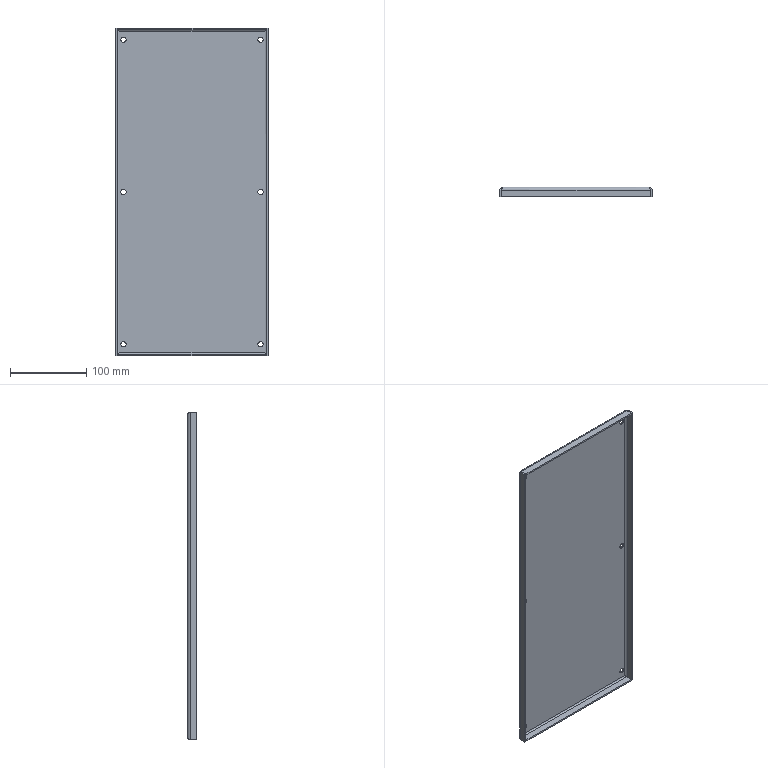Component | SolidWorks | BaseAssembly-1_BaseCover-1 | 1 solid | 50 faces | volume 193280 mm3 | plane 22 | cylinder 20 | spline 8 | commonest cylinder face diameters 7 x12 4 x4 8 x4